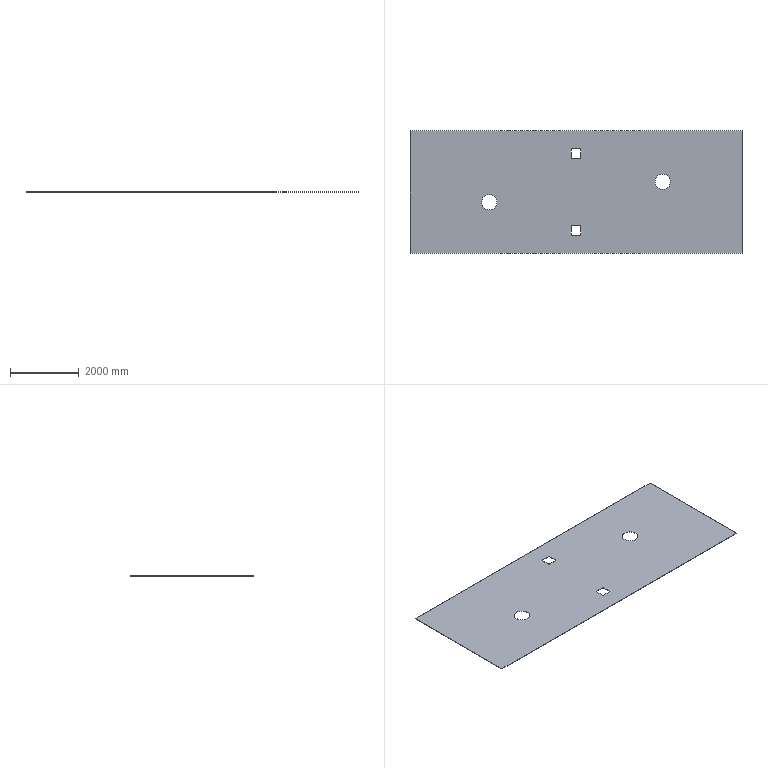Component | SolidWorks | Platform-1 | 1 solid | 26 faces | box 9690 x 3580 x 10 mm | volume 342054589 mm3 | plane 14 | cylinder 12 | commonest cylinder face diameters 60 x8 450 x4 | material Plain Carbon Steel
STEP:
#1=COLOUR_RGB('',0.7922,0.8196,0.9333);
#2=FILL_AREA_STYLE_COLOUR('',#1);
#3=FILL_AREA_STYLE('',(#2));
#4=SURFACE_STYLE_FILL_AREA(#3);
#5=SURFACE_SIDE_STYLE('',(#4));
#6=SURFACE_STYLE_USAGE(.BOTH.,#5);
#7=PRESENTATION_STYLE_ASSIGNMENT((#6));
#8=CARTESIAN_POINT('',(157.197,66.784,219.527));
#9=VERTEX_POINT('',#8);
#10=CARTESIAN_POINT('',(157.197,49.068,219.527));
#11=VERTEX_POINT('',#10);
#12=CARTESIAN_POINT('',(157.197,57.926,219.527));
#13=DIRECTION('',(0.,-0.,1.));
#14=DIRECTION('',(0.,-1.,-0.));
#15=AXIS2_PLACEMENT_3D('',#12,#13,#14);
#16=CIRCLE('',#15,8.858);
#17=EDGE_CURVE('',#9,#11,#16,.T.);
#18=ORIENTED_EDGE('',*,*,#17,.F.);
#19=CARTESIAN_POINT('',(157.197,66.784,219.92));
#20=VERTEX_POINT('',#19);
#21=CARTESIAN_POINT('',(157.197,66.784,219.527));
#22=DIRECTION('',(0.,-0.,1.));
#23=VECTOR('',#22,39.37);
#24=LINE('',#21,#23);
#25=EDGE_CURVE('',#9,#20,#24,.T.);
#26=ORIENTED_EDGE('',*,*,#25,.T.);
#27=CARTESIAN_POINT('',(157.197,49.068,219.92));
#28=VERTEX_POINT('',#27);
#29=CARTESIAN_POINT('',(157.197,57.926,219.92));
#30=DIRECTION('',(0.,-0.,1.));
#31=DIRECTION('',(0.,-1.,-0.));
#32=AXIS2_PLACEMENT_3D('',#29,#30,#31);
#33=CIRCLE('',#32,8.858);
#34=EDGE_CURVE('',#20,#28,#33,.T.);
#35=ORIENTED_EDGE('',*,*,#34,.T.);
#36=CARTESIAN_POINT('',(157.197,49.068,219.527));
#37=DIRECTION('',(0.,-0.,1.));
#38=VECTOR('',#37,39.37);
#39=LINE('',#36,#38);
#40=EDGE_CURVE('',#11,#28,#39,.T.);
#41=ORIENTED_EDGE('',*,*,#40,.F.);
#42=EDGE_LOOP('',(#18,#26,#35,#41));
#43=FACE_OUTER_BOUND('',#42,.T.);
#44=CARTESIAN_POINT('',(157.197,57.926,219.527));
#45=DIRECTION('',(0.,-0.,1.));
#46=DIRECTION('',(0.,-1.,-0.));
#47=AXIS2_PLACEMENT_3D('',#44,#45,#46);
#48=CYLINDRICAL_SURFACE('',#47,8.858);
#49=ADVANCED_FACE('',(#43),#48,.F.);
#50=CARTESIAN_POINT('',(-42.016,43.162,219.527));
#51=VERTEX_POINT('',#50);
#52=CARTESIAN_POINT('',(-42.016,25.446,219.527));
#53=VERTEX_POINT('',#52);
#54=CARTESIAN_POINT('',(-42.016,34.304,219.527));
#55=DIRECTION('',(0.,-0.,1.));
#56=DIRECTION('',(0.,-1.,-0.));
#57=AXIS2_PLACEMENT_3D('',#54,#55,#56);
#58=CIRCLE('',#57,8.858);
#59=EDGE_CURVE('',#51,#53,#58,.T.);
#60=ORIENTED_EDGE('',*,*,#59,.F.);
#61=CARTESIAN_POINT('',(-42.016,43.162,219.92));
#62=VERTEX_POINT('',#61);
#63=CARTESIAN_POINT('',(-42.016,43.162,219.527));
#64=DIRECTION('',(0.,-0.,1.));
#65=VECTOR('',#64,39.37);
#66=LINE('',#63,#65);
#67=EDGE_CURVE('',#51,#62,#66,.T.);
#68=ORIENTED_EDGE('',*,*,#67,.T.);
#69=CARTESIAN_POINT('',(-42.016,25.446,219.92));
#70=VERTEX_POINT('',#69);
#71=CARTESIAN_POINT('',(-42.016,34.304,219.92));
#72=DIRECTION('',(0.,-0.,1.));
#73=DIRECTION('',(0.,-1.,-0.));
#74=AXIS2_PLACEMENT_3D('',#71,#72,#73);
#75=CIRCLE('',#74,8.858);
#76=EDGE_CURVE('',#62,#70,#75,.T.);
#77=ORIENTED_EDGE('',*,*,#76,.T.);
#78=CARTESIAN_POINT('',(-42.016,25.446,219.527));
#79=DIRECTION('',(0.,-0.,1.));
#80=VECTOR('',#79,39.37);
#81=LINE('',#78,#80);
#82=EDGE_CURVE('',#53,#70,#81,.T.);
#83=ORIENTED_EDGE('',*,*,#82,.F.);
#84=EDGE_LOOP('',(#60,#68,#77,#83));
#85=FACE_OUTER_BOUND('',#84,.T.);
#86=CARTESIAN_POINT('',(-42.016,34.304,219.527));
#87=DIRECTION('',(0.,-0.,1.));
#88=DIRECTION('',(0.,-1.,-0.));
#89=AXIS2_PLACEMENT_3D('',#86,#87,#88);
#90=CYLINDRICAL_SURFACE('',#89,8.858);
#91=ADVANCED_FACE('',(#85),#90,.F.);
#92=CARTESIAN_POINT('',(248.339,-24.357,219.92));
#93=VERTEX_POINT('',#92);
#94=CARTESIAN_POINT('',(248.339,116.588,219.92));
#95=VERTEX_POINT('',#94);
#96=CARTESIAN_POINT('',(248.339,116.588,219.92));
#97=DIRECTION('',(0.,1.,0.));
#98=VECTOR('',#97,39.37);
#99=LINE('',#96,#98);
#100=EDGE_CURVE('',#93,#95,#99,.T.);
#101=ORIENTED_EDGE('',*,*,#100,.F.);
#102=CARTESIAN_POINT('',(248.339,-24.357,219.527));
#103=VERTEX_POINT('',#102);
#104=CARTESIAN_POINT('',(248.339,-24.357,219.527));
#105=DIRECTION('',(0.,-0.,1.));
#106=VECTOR('',#105,39.37);
#107=LINE('',#104,#106);
#108=EDGE_CURVE('',#103,#93,#107,.T.);
#109=ORIENTED_EDGE('',*,*,#108,.F.);
#110=CARTESIAN_POINT('',(248.339,116.588,219.527));
#111=VERTEX_POINT('',#110);
#112=CARTESIAN_POINT('',(248.339,116.588,219.527));
#113=DIRECTION('',(0.,1.,0.));
#114=VECTOR('',#113,39.37);
#115=LINE('',#112,#114);
#116=EDGE_CURVE('',#103,#111,#115,.T.);
#117=ORIENTED_EDGE('',*,*,#116,.T.);
#118=CARTESIAN_POINT('',(248.339,116.588,219.527));
#119=DIRECTION('',(0.,-0.,1.));
#120=VECTOR('',#119,39.37);
#121=LINE('',#118,#120);
#122=EDGE_CURVE('',#111,#95,#121,.T.);
#123=ORIENTED_EDGE('',*,*,#122,.T.);
#124=EDGE_LOOP('',(#101,#109,#117,#123));
#125=FACE_OUTER_BOUND('',#124,.T.);
#126=CARTESIAN_POINT('',(248.339,116.588,219.527));
#127=DIRECTION('',(1.,0.,0.));
#128=DIRECTION('',(0.,1.,0.));
#129=AXIS2_PLACEMENT_3D('',#126,#127,#128);
#130=PLANE('',#129);
#131=ADVANCED_FACE('',(#125),#130,.T.);
#132=CARTESIAN_POINT('',(-133.157,-24.357,219.92));
#133=VERTEX_POINT('',#132);
#134=CARTESIAN_POINT('',(-133.157,-24.357,219.92));
#135=DIRECTION('',(1.,0.,0.));
#136=VECTOR('',#135,39.37);
#137=LINE('',#134,#136);
#138=EDGE_CURVE('',#133,#93,#137,.T.);
#139=ORIENTED_EDGE('',*,*,#138,.F.);
#140=CARTESIAN_POINT('',(-133.157,-24.357,219.527));
#141=VERTEX_POINT('',#140);
#142=CARTESIAN_POINT('',(-133.157,-24.357,219.527));
#143=DIRECTION('',(0.,-0.,1.));
#144=VECTOR('',#143,39.37);
#145=LINE('',#142,#144);
#146=EDGE_CURVE('',#141,#133,#145,.T.);
#147=ORIENTED_EDGE('',*,*,#146,.F.);
#148=CARTESIAN_POINT('',(-133.157,-24.357,219.527));
#149=DIRECTION('',(1.,0.,0.));
#150=VECTOR('',#149,39.37);
#151=LINE('',#148,#150);
#152=EDGE_CURVE('',#141,#103,#151,.T.);
#153=ORIENTED_EDGE('',*,*,#152,.T.);
#154=ORIENTED_EDGE('',*,*,#108,.T.);
#155=EDGE_LOOP('',(#139,#147,#153,#154));
#156=FACE_OUTER_BOUND('',#155,.T.);
#157=CARTESIAN_POINT('',(-133.157,-24.357,219.527));
#158=DIRECTION('',(0.,-1.,-0.));
#159=DIRECTION('',(1.,0.,0.));
#160=AXIS2_PLACEMENT_3D('',#157,#158,#159);
#161=PLANE('',#160);
#162=ADVANCED_FACE('',(#156),#161,.T.);
#163=CARTESIAN_POINT('',(-133.157,116.588,219.92));
#164=VERTEX_POINT('',#163);
#165=CARTESIAN_POINT('',(-133.157,116.588,219.92));
#166=DIRECTION('',(0.,-1.,-0.));
#167=VECTOR('',#166,39.37);
#168=LINE('',#165,#167);
#169=EDGE_CURVE('',#164,#133,#168,.T.);
#170=ORIENTED_EDGE('',*,*,#169,.F.);
#171=CARTESIAN_POINT('',(-133.157,116.588,219.527));
#172=VERTEX_POINT('',#171);
#173=CARTESIAN_POINT('',(-133.157,116.588,219.527));
#174=DIRECTION('',(0.,-0.,1.));
#175=VECTOR('',#174,39.37);
#176=LINE('',#173,#175);
#177=EDGE_CURVE('',#172,#164,#176,.T.);
#178=ORIENTED_EDGE('',*,*,#177,.F.);
#179=CARTESIAN_POINT('',(-133.157,116.588,219.527));
#180=DIRECTION('',(0.,-1.,-0.));
#181=VECTOR('',#180,39.37);
#182=LINE('',#179,#181);
#183=EDGE_CURVE('',#172,#141,#182,.T.);
#184=ORIENTED_EDGE('',*,*,#183,.T.);
#185=ORIENTED_EDGE('',*,*,#146,.T.);
#186=EDGE_LOOP('',(#170,#178,#184,#185));
#187=FACE_OUTER_BOUND('',#186,.T.);
#188=CARTESIAN_POINT('',(-133.157,116.588,219.527));
#189=DIRECTION('',(-1.,0.,0.));
#190=DIRECTION('',(0.,-1.,-0.));
#191=AXIS2_PLACEMENT_3D('',#188,#189,#190);
#192=PLANE('',#191);
#193=ADVANCED_FACE('',(#187),#192,.T.);
#194=CARTESIAN_POINT('',(-133.157,116.588,219.92));
#195=DIRECTION('',(-1.,0.,0.));
#196=VECTOR('',#195,39.37);
#197=LINE('',#194,#196);
#198=EDGE_CURVE('',#95,#164,#197,.T.);
#199=ORIENTED_EDGE('',*,*,#198,.F.);
#200=ORIENTED_EDGE('',*,*,#122,.F.);
#201=CARTESIAN_POINT('',(-133.157,116.588,219.527));
#202=DIRECTION('',(-1.,0.,0.));
#203=VECTOR('',#202,39.37);
#204=LINE('',#201,#203);
#205=EDGE_CURVE('',#111,#172,#204,.T.);
#206=ORIENTED_EDGE('',*,*,#205,.T.);
#207=ORIENTED_EDGE('',*,*,#177,.T.);
#208=EDGE_LOOP('',(#199,#200,#206,#207));
#209=FACE_OUTER_BOUND('',#208,.T.);
#210=CARTESIAN_POINT('',(-133.157,116.588,219.527));
#211=DIRECTION('',(0.,1.,0.));
#212=DIRECTION('',(-1.,0.,0.));
#213=AXIS2_PLACEMENT_3D('',#210,#211,#212);
#214=PLANE('',#213);
#215=ADVANCED_FACE('',(#209),#214,.T.);
#216=CARTESIAN_POINT('',(62.118,7.926,219.527));
#217=VERTEX_POINT('',#216);
#218=CARTESIAN_POINT('',(53.063,7.926,219.527));
#219=VERTEX_POINT('',#218);
#220=CARTESIAN_POINT('',(53.063,7.926,219.527));
#221=DIRECTION('',(-1.,0.,0.));
#222=VECTOR('',#221,39.37);
#223=LINE('',#220,#222);
#224=EDGE_CURVE('',#217,#219,#223,.T.);
#225=ORIENTED_EDGE('',*,*,#224,.T.);
#226=CARTESIAN_POINT('',(51.882,6.745,219.527));
#227=VERTEX_POINT('',#226);
#228=CARTESIAN_POINT('',(53.063,6.745,219.527));
#229=DIRECTION('',(0.,-0.,1.));
#230=DIRECTION('',(0.,1.,0.));
#231=AXIS2_PLACEMENT_3D('',#228,#229,#230);
#232=CIRCLE('',#231,1.181);
#233=EDGE_CURVE('',#219,#227,#232,.T.);
#234=ORIENTED_EDGE('',*,*,#233,.T.);
#235=CARTESIAN_POINT('',(51.882,-2.31,219.527));
#236=VERTEX_POINT('',#235);
#237=CARTESIAN_POINT('',(51.882,-2.31,219.527));
#238=DIRECTION('',(-0.,-1.,-0.));
#239=VECTOR('',#238,39.37);
#240=LINE('',#237,#239);
#241=EDGE_CURVE('',#227,#236,#240,.T.);
#242=ORIENTED_EDGE('',*,*,#241,.T.);
#243=CARTESIAN_POINT('',(53.063,-3.491,219.527));
#244=VERTEX_POINT('',#243);
#245=CARTESIAN_POINT('',(53.063,-2.31,219.527));
#246=DIRECTION('',(0.,-0.,1.));
#247=DIRECTION('',(0.,1.,0.));
#248=AXIS2_PLACEMENT_3D('',#245,#246,#247);
#249=CIRCLE('',#248,1.181);
#250=EDGE_CURVE('',#236,#244,#249,.T.);
#251=ORIENTED_EDGE('',*,*,#250,.T.);
#252=CARTESIAN_POINT('',(62.118,-3.491,219.527));
#253=VERTEX_POINT('',#252);
#254=CARTESIAN_POINT('',(53.063,-3.491,219.527));
#255=DIRECTION('',(1.,0.,0.));
#256=VECTOR('',#255,39.37);
#257=LINE('',#254,#256);
#258=EDGE_CURVE('',#244,#253,#257,.T.);
#259=ORIENTED_EDGE('',*,*,#258,.T.);
#260=CARTESIAN_POINT('',(63.299,-2.31,219.527));
#261=VERTEX_POINT('',#260);
#262=CARTESIAN_POINT('',(62.118,-2.31,219.527));
#263=DIRECTION('',(0.,-0.,1.));
#264=DIRECTION('',(0.,-1.,0.));
#265=AXIS2_PLACEMENT_3D('',#262,#263,#264);
#266=CIRCLE('',#265,1.181);
#267=EDGE_CURVE('',#253,#261,#266,.T.);
#268=ORIENTED_EDGE('',*,*,#267,.T.);
#269=CARTESIAN_POINT('',(63.299,6.745,219.527));
#270=VERTEX_POINT('',#269);
#271=CARTESIAN_POINT('',(63.299,-2.31,219.527));
#272=DIRECTION('',(0.,1.,0.));
#273=VECTOR('',#272,39.37);
#274=LINE('',#271,#273);
#275=EDGE_CURVE('',#261,#270,#274,.T.);
#276=ORIENTED_EDGE('',*,*,#275,.T.);
#277=CARTESIAN_POINT('',(62.118,6.745,219.527));
#278=DIRECTION('',(0.,-0.,1.));
#279=DIRECTION('',(0.,1.,0.));
#280=AXIS2_PLACEMENT_3D('',#277,#278,#279);
#281=CIRCLE('',#280,1.181);
#282=EDGE_CURVE('',#270,#217,#281,.T.);
#283=ORIENTED_EDGE('',*,*,#282,.T.);
#284=EDGE_LOOP('',(#225,#234,#242,#251,#259,#268,#276,#283));
#285=FACE_BOUND('',#284,.T.);
#286=CARTESIAN_POINT('',(51.882,94.54,219.527));
#287=VERTEX_POINT('',#286);
#288=CARTESIAN_POINT('',(51.882,85.485,219.527));
#289=VERTEX_POINT('',#288);
#290=CARTESIAN_POINT('',(51.882,94.54,219.527));
#291=DIRECTION('',(0.,-1.,-0.));
#292=VECTOR('',#291,39.37);
#293=LINE('',#290,#292);
#294=EDGE_CURVE('',#287,#289,#293,.T.);
#295=ORIENTED_EDGE('',*,*,#294,.T.);
#296=CARTESIAN_POINT('',(53.063,84.304,219.527));
#297=VERTEX_POINT('',#296);
#298=CARTESIAN_POINT('',(53.063,85.485,219.527));
#299=DIRECTION('',(0.,-0.,1.));
#300=DIRECTION('',(0.,-1.,0.));
#301=AXIS2_PLACEMENT_3D('',#298,#299,#300);
#302=CIRCLE('',#301,1.181);
#303=EDGE_CURVE('',#289,#297,#302,.T.);
#304=ORIENTED_EDGE('',*,*,#303,.T.);
#305=CARTESIAN_POINT('',(62.118,84.304,219.527));
#306=VERTEX_POINT('',#305);
#307=CARTESIAN_POINT('',(53.063,84.304,219.527));
#308=DIRECTION('',(1.,0.,0.));
#309=VECTOR('',#308,39.37);
#310=LINE('',#307,#309);
#311=EDGE_CURVE('',#297,#306,#310,.T.);
#312=ORIENTED_EDGE('',*,*,#311,.T.);
#313=CARTESIAN_POINT('',(63.299,85.485,219.527));
#314=VERTEX_POINT('',#313);
#315=CARTESIAN_POINT('',(62.118,85.485,219.527));
#316=DIRECTION('',(0.,-0.,1.));
#317=DIRECTION('',(0.,-1.,0.));
#318=AXIS2_PLACEMENT_3D('',#315,#316,#317);
#319=CIRCLE('',#318,1.181);
#320=EDGE_CURVE('',#306,#314,#319,.T.);
#321=ORIENTED_EDGE('',*,*,#320,.T.);
#322=CARTESIAN_POINT('',(63.299,94.54,219.527));
#323=VERTEX_POINT('',#322);
#324=CARTESIAN_POINT('',(63.299,94.54,219.527));
#325=DIRECTION('',(-0.,1.,0.));
#326=VECTOR('',#325,39.37);
#327=LINE('',#324,#326);
#328=EDGE_CURVE('',#314,#323,#327,.T.);
#329=ORIENTED_EDGE('',*,*,#328,.T.);
#330=CARTESIAN_POINT('',(62.118,95.721,219.527));
#331=VERTEX_POINT('',#330);
#332=CARTESIAN_POINT('',(62.118,94.54,219.527));
#333=DIRECTION('',(0.,-0.,1.));
#334=DIRECTION('',(0.,1.,0.));
#335=AXIS2_PLACEMENT_3D('',#332,#333,#334);
#336=CIRCLE('',#335,1.181);
#337=EDGE_CURVE('',#323,#331,#336,.T.);
#338=ORIENTED_EDGE('',*,*,#337,.T.);
#339=CARTESIAN_POINT('',(53.063,95.721,219.527));
#340=VERTEX_POINT('',#339);
#341=CARTESIAN_POINT('',(53.063,95.721,219.527));
#342=DIRECTION('',(-1.,0.,0.));
#343=VECTOR('',#342,39.37);
#344=LINE('',#341,#343);
#345=EDGE_CURVE('',#331,#340,#344,.T.);
#346=ORIENTED_EDGE('',*,*,#345,.T.);
#347=CARTESIAN_POINT('',(53.063,94.54,219.527));
#348=DIRECTION('',(0.,-0.,1.));
#349=DIRECTION('',(0.,-1.,0.));
#350=AXIS2_PLACEMENT_3D('',#347,#348,#349);
#351=CIRCLE('',#350,1.181);
#352=EDGE_CURVE('',#340,#287,#351,.T.);
#353=ORIENTED_EDGE('',*,*,#352,.T.);
#354=EDGE_LOOP('',(#295,#304,#312,#321,#329,#338,#346,#353));
#355=FACE_BOUND('',#354,.T.);
#356=CARTESIAN_POINT('',(157.197,57.926,219.527));
#357=DIRECTION('',(0.,-0.,1.));
#358=DIRECTION('',(0.,-1.,-0.));
#359=AXIS2_PLACEMENT_3D('',#356,#357,#358);
#360=CIRCLE('',#359,8.858);
#361=EDGE_CURVE('',#11,#9,#360,.T.);
#362=ORIENTED_EDGE('',*,*,#361,.T.);
#363=ORIENTED_EDGE('',*,*,#17,.T.);
#364=EDGE_LOOP('',(#362,#363));
#365=FACE_BOUND('',#364,.T.);
#366=CARTESIAN_POINT('',(-42.016,34.304,219.527));
#367=DIRECTION('',(0.,-0.,1.));
#368=DIRECTION('',(0.,-1.,-0.));
#369=AXIS2_PLACEMENT_3D('',#366,#367,#368);
#370=CIRCLE('',#369,8.858);
#371=EDGE_CURVE('',#53,#51,#370,.T.);
#372=ORIENTED_EDGE('',*,*,#371,.T.);
#373=ORIENTED_EDGE('',*,*,#59,.T.);
#374=EDGE_LOOP('',(#372,#373));
#375=FACE_BOUND('',#374,.T.);
#376=ORIENTED_EDGE('',*,*,#116,.F.);
#377=ORIENTED_EDGE('',*,*,#152,.F.);
#378=ORIENTED_EDGE('',*,*,#183,.F.);
#379=ORIENTED_EDGE('',*,*,#205,.F.);
#380=EDGE_LOOP('',(#376,#377,#378,#379));
#381=FACE_OUTER_BOUND('',#380,.T.);
#382=CARTESIAN_POINT('',(57.591,46.115,219.527));
#383=DIRECTION('',(0.,-0.,1.));
#384=DIRECTION('',(0.,-1.,-0.));
#385=AXIS2_PLACEMENT_3D('',#382,#383,#384);
#386=PLANE('',#385);
#387=ADVANCED_FACE('',(#285,#355,#365,#375,#381),#386,.F.);
#388=CARTESIAN_POINT('',(53.063,7.926,219.92));
#389=VERTEX_POINT('',#388);
#390=CARTESIAN_POINT('',(51.882,6.745,219.92));
#391=VERTEX_POINT('',#390);
#392=CARTESIAN_POINT('',(53.063,6.745,219.92));
#393=DIRECTION('',(0.,-0.,1.));
#394=DIRECTION('',(0.,1.,0.));
#395=AXIS2_PLACEMENT_3D('',#392,#393,#394);
#396=CIRCLE('',#395,1.181);
#397=EDGE_CURVE('',#389,#391,#396,.T.);
#398=ORIENTED_EDGE('',*,*,#397,.F.);
#399=CARTESIAN_POINT('',(62.118,7.926,219.92));
#400=VERTEX_POINT('',#399);
#401=CARTESIAN_POINT('',(53.063,7.926,219.92));
#402=DIRECTION('',(-1.,0.,0.));
#403=VECTOR('',#402,39.37);
#404=LINE('',#401,#403);
#405=EDGE_CURVE('',#400,#389,#404,.T.);
#406=ORIENTED_EDGE('',*,*,#405,.F.);
#407=CARTESIAN_POINT('',(63.299,6.745,219.92));
#408=VERTEX_POINT('',#407);
#409=CARTESIAN_POINT('',(62.118,6.745,219.92));
#410=DIRECTION('',(0.,-0.,1.));
#411=DIRECTION('',(0.,1.,0.));
#412=AXIS2_PLACEMENT_3D('',#409,#410,#411);
#413=CIRCLE('',#412,1.181);
#414=EDGE_CURVE('',#408,#400,#413,.T.);
#415=ORIENTED_EDGE('',*,*,#414,.F.);
#416=CARTESIAN_POINT('',(63.299,-2.31,219.92));
#417=VERTEX_POINT('',#416);
#418=CARTESIAN_POINT('',(63.299,-2.31,219.92));
#419=DIRECTION('',(0.,1.,0.));
#420=VECTOR('',#419,39.37);
#421=LINE('',#418,#420);
#422=EDGE_CURVE('',#417,#408,#421,.T.);
#423=ORIENTED_EDGE('',*,*,#422,.F.);
#424=CARTESIAN_POINT('',(62.118,-3.491,219.92));
#425=VERTEX_POINT('',#424);
#426=CARTESIAN_POINT('',(62.118,-2.31,219.92));
#427=DIRECTION('',(0.,-0.,1.));
#428=DIRECTION('',(0.,-1.,0.));
#429=AXIS2_PLACEMENT_3D('',#426,#427,#428);
#430=CIRCLE('',#429,1.181);
#431=EDGE_CURVE('',#425,#417,#430,.T.);
#432=ORIENTED_EDGE('',*,*,#431,.F.);
#433=CARTESIAN_POINT('',(53.063,-3.491,219.92));
#434=VERTEX_POINT('',#433);
#435=CARTESIAN_POINT('',(53.063,-3.491,219.92));
#436=DIRECTION('',(1.,0.,0.));
#437=VECTOR('',#436,39.37);
#438=LINE('',#435,#437);
#439=EDGE_CURVE('',#434,#425,#438,.T.);
#440=ORIENTED_EDGE('',*,*,#439,.F.);
#441=CARTESIAN_POINT('',(51.882,-2.31,219.92));
#442=VERTEX_POINT('',#441);
#443=CARTESIAN_POINT('',(53.063,-2.31,219.92));
#444=DIRECTION('',(0.,-0.,1.));
#445=DIRECTION('',(0.,1.,0.));
#446=AXIS2_PLACEMENT_3D('',#443,#444,#445);
#447=CIRCLE('',#446,1.181);
#448=EDGE_CURVE('',#442,#434,#447,.T.);
#449=ORIENTED_EDGE('',*,*,#448,.F.);
#450=CARTESIAN_POINT('',(51.882,-2.31,219.92));
#451=DIRECTION('',(-0.,-1.,-0.));
#452=VECTOR('',#451,39.37);
#453=LINE('',#450,#452);
#454=EDGE_CURVE('',#391,#442,#453,.T.);
#455=ORIENTED_EDGE('',*,*,#454,.F.);
#456=EDGE_LOOP('',(#398,#406,#415,#423,#432,#440,#449,#455));
#457=FACE_BOUND('',#456,.T.);
#458=CARTESIAN_POINT('',(51.882,85.485,219.92));
#459=VERTEX_POINT('',#458);
#460=CARTESIAN_POINT('',(53.063,84.304,219.92));
#461=VERTEX_POINT('',#460);
#462=CARTESIAN_POINT('',(53.063,85.485,219.92));
#463=DIRECTION('',(0.,-0.,1.));
#464=DIRECTION('',(0.,-1.,0.));
#465=AXIS2_PLACEMENT_3D('',#462,#463,#464);
#466=CIRCLE('',#465,1.181);
#467=EDGE_CURVE('',#459,#461,#466,.T.);
#468=ORIENTED_EDGE('',*,*,#467,.F.);
#469=CARTESIAN_POINT('',(51.882,94.54,219.92));
#470=VERTEX_POINT('',#469);
#471=CARTESIAN_POINT('',(51.882,94.54,219.92));
#472=DIRECTION('',(0.,-1.,-0.));
#473=VECTOR('',#472,39.37);
#474=LINE('',#471,#473);
#475=EDGE_CURVE('',#470,#459,#474,.T.);
#476=ORIENTED_EDGE('',*,*,#475,.F.);
#477=CARTESIAN_POINT('',(53.063,95.721,219.92));
#478=VERTEX_POINT('',#477);
#479=CARTESIAN_POINT('',(53.063,94.54,219.92));
#480=DIRECTION('',(0.,-0.,1.));
#481=DIRECTION('',(0.,-1.,0.));
#482=AXIS2_PLACEMENT_3D('',#479,#480,#481);
#483=CIRCLE('',#482,1.181);
#484=EDGE_CURVE('',#478,#470,#483,.T.);
#485=ORIENTED_EDGE('',*,*,#484,.F.);
#486=CARTESIAN_POINT('',(62.118,95.721,219.92));
#487=VERTEX_POINT('',#486);
#488=CARTESIAN_POINT('',(53.063,95.721,219.92));
#489=DIRECTION('',(-1.,0.,0.));
#490=VECTOR('',#489,39.37);
#491=LINE('',#488,#490);
#492=EDGE_CURVE('',#487,#478,#491,.T.);
#493=ORIENTED_EDGE('',*,*,#492,.F.);
#494=CARTESIAN_POINT('',(63.299,94.54,219.92));
#495=VERTEX_POINT('',#494);
#496=CARTESIAN_POINT('',(62.118,94.54,219.92));
#497=DIRECTION('',(0.,-0.,1.));
#498=DIRECTION('',(0.,1.,0.));
#499=AXIS2_PLACEMENT_3D('',#496,#497,#498);
#500=CIRCLE('',#499,1.181);
#501=EDGE_CURVE('',#495,#487,#500,.T.);
#502=ORIENTED_EDGE('',*,*,#501,.F.);
#503=CARTESIAN_POINT('',(63.299,85.485,219.92));
#504=VERTEX_POINT('',#503);
#505=CARTESIAN_POINT('',(63.299,94.54,219.92));
#506=DIRECTION('',(-0.,1.,0.));
#507=VECTOR('',#506,39.37);
#508=LINE('',#505,#507);
#509=EDGE_CURVE('',#504,#495,#508,.T.);
#510=ORIENTED_EDGE('',*,*,#509,.F.);
#511=CARTESIAN_POINT('',(62.118,84.304,219.92));
#512=VERTEX_POINT('',#511);
#513=CARTESIAN_POINT('',(62.118,85.485,219.92));
#514=DIRECTION('',(0.,-0.,1.));
#515=DIRECTION('',(0.,-1.,0.));
#516=AXIS2_PLACEMENT_3D('',#513,#514,#515);
#517=CIRCLE('',#516,1.181);
#518=EDGE_CURVE('',#512,#504,#517,.T.);
#519=ORIENTED_EDGE('',*,*,#518,.F.);
#520=CARTESIAN_POINT('',(53.063,84.304,219.92));
#521=DIRECTION('',(1.,0.,0.));
#522=VECTOR('',#521,39.37);
#523=LINE('',#520,#522);
#524=EDGE_CURVE('',#461,#512,#523,.T.);
#525=ORIENTED_EDGE('',*,*,#524,.F.);
#526=EDGE_LOOP('',(#468,#476,#485,#493,#502,#510,#519,#525));
#527=FACE_BOUND('',#526,.T.);
#528=CARTESIAN_POINT('',(157.197,57.926,219.92));
#529=DIRECTION('',(0.,-0.,1.));
#530=DIRECTION('',(0.,-1.,-0.));
#531=AXIS2_PLACEMENT_3D('',#528,#529,#530);
#532=CIRCLE('',#531,8.858);
#533=EDGE_CURVE('',#28,#20,#532,.T.);
#534=ORIENTED_EDGE('',*,*,#533,.F.);
#535=ORIENTED_EDGE('',*,*,#34,.F.);
#536=EDGE_LOOP('',(#534,#535));
#537=FACE_BOUND('',#536,.T.);
#538=CARTESIAN_POINT('',(-42.016,34.304,219.92));
#539=DIRECTION('',(0.,-0.,1.));
#540=DIRECTION('',(0.,-1.,-0.));
#541=AXIS2_PLACEMENT_3D('',#538,#539,#540);
#542=CIRCLE('',#541,8.858);
#543=EDGE_CURVE('',#70,#62,#542,.T.);
#544=ORIENTED_EDGE('',*,*,#543,.F.);
#545=ORIENTED_EDGE('',*,*,#76,.F.);
#546=EDGE_LOOP('',(#544,#545));
#547=FACE_BOUND('',#546,.T.);
#548=ORIENTED_EDGE('',*,*,#100,.T.);
#549=ORIENTED_EDGE('',*,*,#198,.T.);
#550=ORIENTED_EDGE('',*,*,#169,.T.);
#551=ORIENTED_EDGE('',*,*,#138,.T.);
#552=EDGE_LOOP('',(#548,#549,#550,#551));
#553=FACE_OUTER_BOUND('',#552,.T.);
#554=CARTESIAN_POINT('',(57.591,46.115,219.92));
#555=DIRECTION('',(0.,-0.,1.));
#556=DIRECTION('',(0.,-1.,-0.));
#557=AXIS2_PLACEMENT_3D('',#554,#555,#556);
#558=PLANE('',#557);
#559=ADVANCED_FACE('',(#457,#527,#537,#547,#553),#558,.T.);
#560=ORIENTED_EDGE('',*,*,#67,.F.);
#561=ORIENTED_EDGE('',*,*,#371,.F.);
#562=ORIENTED_EDGE('',*,*,#82,.T.);
#563=ORIENTED_EDGE('',*,*,#543,.T.);
#564=EDGE_LOOP('',(#560,#561,#562,#563));
#565=FACE_OUTER_BOUND('',#564,.T.);
#566=CARTESIAN_POINT('',(-42.016,34.304,219.527));
#567=DIRECTION('',(0.,-0.,1.));
#568=DIRECTION('',(0.,-1.,-0.));
#569=AXIS2_PLACEMENT_3D('',#566,#567,#568);
#570=CYLINDRICAL_SURFACE('',#569,8.858);
#571=ADVANCED_FACE('',(#565),#570,.F.);
#572=ORIENTED_EDGE('',*,*,#25,.F.);
#573=ORIENTED_EDGE('',*,*,#361,.F.);
#574=ORIENTED_EDGE('',*,*,#40,.T.);
#575=ORIENTED_EDGE('',*,*,#533,.T.);
#576=EDGE_LOOP('',(#572,#573,#574,#575));
#577=FACE_OUTER_BOUND('',#576,.T.);
#578=CARTESIAN_POINT('',(157.197,57.926,219.527));
#579=DIRECTION('',(0.,-0.,1.));
#580=DIRECTION('',(0.,-1.,-0.));
#581=AXIS2_PLACEMENT_3D('',#578,#579,#580);
#582=CYLINDRICAL_SURFACE('',#581,8.858);
#583=ADVANCED_FACE('',(#577),#582,.F.);
#584=ORIENTED_EDGE('',*,*,#467,.T.);
#585=CARTESIAN_POINT('',(53.063,84.304,219.527));
#586=DIRECTION('',(0.,-0.,1.));
#587=VECTOR('',#586,39.37);
#588=LINE('',#585,#587);
#589=EDGE_CURVE('',#297,#461,#588,.T.);
#590=ORIENTED_EDGE('',*,*,#589,.F.);
#591=ORIENTED_EDGE('',*,*,#303,.F.);
#592=CARTESIAN_POINT('',(51.882,85.485,219.527));
#593=DIRECTION('',(0.,-0.,1.));
#594=VECTOR('',#593,39.37);
#595=LINE('',#592,#594);
#596=EDGE_CURVE('',#289,#459,#595,.T.);
#597=ORIENTED_EDGE('',*,*,#596,.T.);
#598=EDGE_LOOP('',(#584,#590,#591,#597));
#599=FACE_OUTER_BOUND('',#598,.T.);
#600=CARTESIAN_POINT('',(53.063,85.485,219.527));
#601=DIRECTION('',(0.,-0.,1.));
#602=DIRECTION('',(0.,-1.,0.));
#603=AXIS2_PLACEMENT_3D('',#600,#601,#602);
#604=CYLINDRICAL_SURFACE('',#603,1.181);
#605=ADVANCED_FACE('',(#599),#604,.F.);
#606=ORIENTED_EDGE('',*,*,#475,.T.);
#607=ORIENTED_EDGE('',*,*,#596,.F.);
#608=ORIENTED_EDGE('',*,*,#294,.F.);
#609=CARTESIAN_POINT('',(51.882,94.54,219.527));
#610=DIRECTION('',(0.,-0.,1.));
#611=VECTOR('',#610,39.37);
#612=LINE('',#609,#611);
#613=EDGE_CURVE('',#287,#470,#612,.T.);
#614=ORIENTED_EDGE('',*,*,#613,.T.);
#615=EDGE_LOOP('',(#606,#607,#608,#614));
#616=FACE_OUTER_BOUND('',#615,.T.);
#617=CARTESIAN_POINT('',(51.882,94.54,219.527));
#618=DIRECTION('',(-1.,-0.,-0.));
#619=DIRECTION('',(0.,-1.,-0.));
#620=AXIS2_PLACEMENT_3D('',#617,#618,#619);
#621=PLANE('',#620);
#622=ADVANCED_FACE('',(#616),#621,.F.);
#623=ORIENTED_EDGE('',*,*,#484,.T.);
#624=ORIENTED_EDGE('',*,*,#613,.F.);
#625=ORIENTED_EDGE('',*,*,#352,.F.);
#626=CARTESIAN_POINT('',(53.063,95.721,219.527));
#627=DIRECTION('',(0.,-0.,1.));
#628=VECTOR('',#627,39.37);
#629=LINE('',#626,#628);
#630=EDGE_CURVE('',#340,#478,#629,.T.);
#631=ORIENTED_EDGE('',*,*,#630,.T.);
#632=EDGE_LOOP('',(#623,#624,#625,#631));
#633=FACE_OUTER_BOUND('',#632,.T.);
#634=CARTESIAN_POINT('',(53.063,94.54,219.527));
#635=DIRECTION('',(0.,-0.,1.));
#636=DIRECTION('',(0.,-1.,0.));
#637=AXIS2_PLACEMENT_3D('',#634,#635,#636);
#638=CYLINDRICAL_SURFACE('',#637,1.181);
#639=ADVANCED_FACE('',(#633),#638,.F.);
#640=ORIENTED_EDGE('',*,*,#492,.T.);
#641=ORIENTED_EDGE('',*,*,#630,.F.);
#642=ORIENTED_EDGE('',*,*,#345,.F.);
#643=CARTESIAN_POINT('',(62.118,95.721,219.527));
#644=DIRECTION('',(0.,-0.,1.));
#645=VECTOR('',#644,39.37);
#646=LINE('',#643,#645);
#647=EDGE_CURVE('',#331,#487,#646,.T.);
#648=ORIENTED_EDGE('',*,*,#647,.T.);
#649=EDGE_LOOP('',(#640,#641,#642,#648));
#650=FACE_OUTER_BOUND('',#649,.T.);
#651=CARTESIAN_POINT('',(53.063,95.721,219.527));
#652=DIRECTION('',(0.,1.,0.));
#653=DIRECTION('',(-1.,0.,0.));
#654=AXIS2_PLACEMENT_3D('',#651,#652,#653);
#655=PLANE('',#654);
#656=ADVANCED_FACE('',(#650),#655,.F.);
#657=ORIENTED_EDGE('',*,*,#501,.T.);
#658=ORIENTED_EDGE('',*,*,#647,.F.);
#659=ORIENTED_EDGE('',*,*,#337,.F.);
#660=CARTESIAN_POINT('',(63.299,94.54,219.527));
#661=DIRECTION('',(0.,-0.,1.));
#662=VECTOR('',#661,39.37);
#663=LINE('',#660,#662);
#664=EDGE_CURVE('',#323,#495,#663,.T.);
#665=ORIENTED_EDGE('',*,*,#664,.T.);
#666=EDGE_LOOP('',(#657,#658,#659,#665));
#667=FACE_OUTER_BOUND('',#666,.T.);
#668=CARTESIAN_POINT('',(62.118,94.54,219.527));
#669=DIRECTION('',(0.,-0.,1.));
#670=DIRECTION('',(0.,-1.,0.));
#671=AXIS2_PLACEMENT_3D('',#668,#669,#670);
#672=CYLINDRICAL_SURFACE('',#671,1.181);
#673=ADVANCED_FACE('',(#667),#672,.F.);
#674=ORIENTED_EDGE('',*,*,#509,.T.);
#675=ORIENTED_EDGE('',*,*,#664,.F.);
#676=ORIENTED_EDGE('',*,*,#328,.F.);
#677=CARTESIAN_POINT('',(63.299,85.485,219.527));
#678=DIRECTION('',(0.,-0.,1.));
#679=VECTOR('',#678,39.37);
#680=LINE('',#677,#679);
#681=EDGE_CURVE('',#314,#504,#680,.T.);
#682=ORIENTED_EDGE('',*,*,#681,.T.);
#683=EDGE_LOOP('',(#674,#675,#676,#682));
#684=FACE_OUTER_BOUND('',#683,.T.);
#685=CARTESIAN_POINT('',(63.299,94.54,219.527));
#686=DIRECTION('',(1.,0.,0.));
#687=DIRECTION('',(-0.,1.,0.));
#688=AXIS2_PLACEMENT_3D('',#685,#686,#687);
#689=PLANE('',#688);
#690=ADVANCED_FACE('',(#684),#689,.F.);
#691=ORIENTED_EDGE('',*,*,#518,.T.);
#692=ORIENTED_EDGE('',*,*,#681,.F.);
#693=ORIENTED_EDGE('',*,*,#320,.F.);
#694=CARTESIAN_POINT('',(62.118,84.304,219.527));
#695=DIRECTION('',(0.,-0.,1.));
#696=VECTOR('',#695,39.37);
#697=LINE('',#694,#696);
#698=EDGE_CURVE('',#306,#512,#697,.T.);
#699=ORIENTED_EDGE('',*,*,#698,.T.);
#700=EDGE_LOOP('',(#691,#692,#693,#699));
#701=FACE_OUTER_BOUND('',#700,.T.);
#702=CARTESIAN_POINT('',(62.118,85.485,219.527));
#703=DIRECTION('',(0.,-0.,1.));
#704=DIRECTION('',(0.,-1.,0.));
#705=AXIS2_PLACEMENT_3D('',#702,#703,#704);
#706=CYLINDRICAL_SURFACE('',#705,1.181);
#707=ADVANCED_FACE('',(#701),#706,.F.);
#708=ORIENTED_EDGE('',*,*,#524,.T.);
#709=ORIENTED_EDGE('',*,*,#698,.F.);
#710=ORIENTED_EDGE('',*,*,#311,.F.);
#711=ORIENTED_EDGE('',*,*,#589,.T.);
#712=EDGE_LOOP('',(#708,#709,#710,#711));
#713=FACE_OUTER_BOUND('',#712,.T.);
#714=CARTESIAN_POINT('',(53.063,84.304,219.527));
#715=DIRECTION('',(0.,-1.,-0.));
#716=DIRECTION('',(1.,0.,0.));
#717=AXIS2_PLACEMENT_3D('',#714,#715,#716);
#718=PLANE('',#717);
#719=ADVANCED_FACE('',(#713),#718,.F.);
#720=ORIENTED_EDGE('',*,*,#397,.T.);
#721=CARTESIAN_POINT('',(51.882,6.745,219.527));
#722=DIRECTION('',(0.,-0.,1.));
#723=VECTOR('',#722,39.37);
#724=LINE('',#721,#723);
#725=EDGE_CURVE('',#227,#391,#724,.T.);
#726=ORIENTED_EDGE('',*,*,#725,.F.);
#727=ORIENTED_EDGE('',*,*,#233,.F.);
#728=CARTESIAN_POINT('',(53.063,7.926,219.527));
#729=DIRECTION('',(0.,-0.,1.));
#730=VECTOR('',#729,39.37);
#731=LINE('',#728,#730);
#732=EDGE_CURVE('',#219,#389,#731,.T.);
#733=ORIENTED_EDGE('',*,*,#732,.T.);
#734=EDGE_LOOP('',(#720,#726,#727,#733));
#735=FACE_OUTER_BOUND('',#734,.T.);
#736=CARTESIAN_POINT('',(53.063,6.745,219.527));
#737=DIRECTION('',(0.,-0.,1.));
#738=DIRECTION('',(0.,-1.,0.));
#739=AXIS2_PLACEMENT_3D('',#736,#737,#738);
#740=CYLINDRICAL_SURFACE('',#739,1.181);
#741=ADVANCED_FACE('',(#735),#740,.F.);
#742=ORIENTED_EDGE('',*,*,#405,.T.);
#743=ORIENTED_EDGE('',*,*,#732,.F.);
#744=ORIENTED_EDGE('',*,*,#224,.F.);
#745=CARTESIAN_POINT('',(62.118,7.926,219.527));
#746=DIRECTION('',(0.,-0.,1.));
#747=VECTOR('',#746,39.37);
#748=LINE('',#745,#747);
#749=EDGE_CURVE('',#217,#400,#748,.T.);
#750=ORIENTED_EDGE('',*,*,#749,.T.);
#751=EDGE_LOOP('',(#742,#743,#744,#750));
#752=FACE_OUTER_BOUND('',#751,.T.);
#753=CARTESIAN_POINT('',(53.063,7.926,219.527));
#754=DIRECTION('',(0.,1.,0.));
#755=DIRECTION('',(-1.,0.,0.));
#756=AXIS2_PLACEMENT_3D('',#753,#754,#755);
#757=PLANE('',#756);
#758=ADVANCED_FACE('',(#752),#757,.F.);
#759=ORIENTED_EDGE('',*,*,#414,.T.);
#760=ORIENTED_EDGE('',*,*,#749,.F.);
#761=ORIENTED_EDGE('',*,*,#282,.F.);
#762=CARTESIAN_POINT('',(63.299,6.745,219.527));
#763=DIRECTION('',(0.,-0.,1.));
#764=VECTOR('',#763,39.37);
#765=LINE('',#762,#764);
#766=EDGE_CURVE('',#270,#408,#765,.T.);
#767=ORIENTED_EDGE('',*,*,#766,.T.);
#768=EDGE_LOOP('',(#759,#760,#761,#767));
#769=FACE_OUTER_BOUND('',#768,.T.);
#770=CARTESIAN_POINT('',(62.118,6.745,219.527));
#771=DIRECTION('',(0.,-0.,1.));
#772=DIRECTION('',(0.,-1.,0.));
#773=AXIS2_PLACEMENT_3D('',#770,#771,#772);
#774=CYLINDRICAL_SURFACE('',#773,1.181);
#775=ADVANCED_FACE('',(#769),#774,.F.);
#776=ORIENTED_EDGE('',*,*,#422,.T.);
#777=ORIENTED_EDGE('',*,*,#766,.F.);
#778=ORIENTED_EDGE('',*,*,#275,.F.);
#779=CARTESIAN_POINT('',(63.299,-2.31,219.527));
#780=DIRECTION('',(0.,-0.,1.));
#781=VECTOR('',#780,39.37);
#782=LINE('',#779,#781);
#783=EDGE_CURVE('',#261,#417,#782,.T.);
#784=ORIENTED_EDGE('',*,*,#783,.T.);
#785=EDGE_LOOP('',(#776,#777,#778,#784));
#786=FACE_OUTER_BOUND('',#785,.T.);
#787=CARTESIAN_POINT('',(63.299,-2.31,219.527));
#788=DIRECTION('',(1.,-0.,-0.));
#789=DIRECTION('',(0.,1.,0.));
#790=AXIS2_PLACEMENT_3D('',#787,#788,#789);
#791=PLANE('',#790);
#792=ADVANCED_FACE('',(#786),#791,.F.);
#793=ORIENTED_EDGE('',*,*,#431,.T.);
#794=ORIENTED_EDGE('',*,*,#783,.F.);
#795=ORIENTED_EDGE('',*,*,#267,.F.);
#796=CARTESIAN_POINT('',(62.118,-3.491,219.527));
#797=DIRECTION('',(0.,-0.,1.));
#798=VECTOR('',#797,39.37);
#799=LINE('',#796,#798);
#800=EDGE_CURVE('',#253,#425,#799,.T.);
#801=ORIENTED_EDGE('',*,*,#800,.T.);
#802=EDGE_LOOP('',(#793,#794,#795,#801));
#803=FACE_OUTER_BOUND('',#802,.T.);
#804=CARTESIAN_POINT('',(62.118,-2.31,219.527));
#805=DIRECTION('',(0.,-0.,1.));
#806=DIRECTION('',(0.,-1.,0.));
#807=AXIS2_PLACEMENT_3D('',#804,#805,#806);
#808=CYLINDRICAL_SURFACE('',#807,1.181);
#809=ADVANCED_FACE('',(#803),#808,.F.);
#810=ORIENTED_EDGE('',*,*,#439,.T.);
#811=ORIENTED_EDGE('',*,*,#800,.F.);
#812=ORIENTED_EDGE('',*,*,#258,.F.);
#813=CARTESIAN_POINT('',(53.063,-3.491,219.527));
#814=DIRECTION('',(0.,-0.,1.));
#815=VECTOR('',#814,39.37);
#816=LINE('',#813,#815);
#817=EDGE_CURVE('',#244,#434,#816,.T.);
#818=ORIENTED_EDGE('',*,*,#817,.T.);
#819=EDGE_LOOP('',(#810,#811,#812,#818));
#820=FACE_OUTER_BOUND('',#819,.T.);
#821=CARTESIAN_POINT('',(53.063,-3.491,219.527));
#822=DIRECTION('',(0.,-1.,-0.));
#823=DIRECTION('',(1.,0.,0.));
#824=AXIS2_PLACEMENT_3D('',#821,#822,#823);
#825=PLANE('',#824);
#826=ADVANCED_FACE('',(#820),#825,.F.);
#827=ORIENTED_EDGE('',*,*,#448,.T.);
#828=ORIENTED_EDGE('',*,*,#817,.F.);
#829=ORIENTED_EDGE('',*,*,#250,.F.);
#830=CARTESIAN_POINT('',(51.882,-2.31,219.527));
#831=DIRECTION('',(0.,-0.,1.));
#832=VECTOR('',#831,39.37);
#833=LINE('',#830,#832);
#834=EDGE_CURVE('',#236,#442,#833,.T.);
#835=ORIENTED_EDGE('',*,*,#834,.T.);
#836=EDGE_LOOP('',(#827,#828,#829,#835));
#837=FACE_OUTER_BOUND('',#836,.T.);
#838=CARTESIAN_POINT('',(53.063,-2.31,219.527));
#839=DIRECTION('',(0.,-0.,1.));
#840=DIRECTION('',(0.,-1.,0.));
#841=AXIS2_PLACEMENT_3D('',#838,#839,#840);
#842=CYLINDRICAL_SURFACE('',#841,1.181);
#843=ADVANCED_FACE('',(#837),#842,.F.);
#844=ORIENTED_EDGE('',*,*,#454,.T.);
#845=ORIENTED_EDGE('',*,*,#834,.F.);
#846=ORIENTED_EDGE('',*,*,#241,.F.);
#847=ORIENTED_EDGE('',*,*,#725,.T.);
#848=EDGE_LOOP('',(#844,#845,#846,#847));
#849=FACE_OUTER_BOUND('',#848,.T.);
#850=CARTESIAN_POINT('',(51.882,-2.31,219.527));
#851=DIRECTION('',(-1.,0.,0.));
#852=DIRECTION('',(-0.,-1.,-0.));
#853=AXIS2_PLACEMENT_3D('',#850,#851,#852);
#854=PLANE('',#853);
#855=ADVANCED_FACE('',(#849),#854,.F.);
#856=CLOSED_SHELL('',(#49,#91,#131,#162,#193,#215,#387,#559,#571,#583,#605,#622,#639,#656,#673,#690,#707,#719,#741,#758,#775,#792,#809,#826,#843,#855));
#857=MANIFOLD_SOLID_BREP('',#856);
#858=STYLED_ITEM('',(#7),#857);
#859=PRESENTATION_LAYER_ASSIGNMENT('','',(#858));
#860=(LENGTH_UNIT()NAMED_UNIT(*)SI_UNIT($,.METRE.));
#861=LENGTH_MEASURE_WITH_UNIT(LENGTH_MEASURE(0.0254),#860);
#862=DIMENSIONAL_EXPONENTS(1.,0.,0.,0.,0.,0.,0.);
#863=(CONVERSION_BASED_UNIT('',#861)LENGTH_UNIT()NAMED_UNIT(#862));
#864=UNCERTAINTY_MEASURE_WITH_UNIT(LENGTH_MEASURE(0.00001),#863,'','');
#865=(NAMED_UNIT(*)PLANE_ANGLE_UNIT()SI_UNIT($,.RADIAN.));
#866=(NAMED_UNIT(*)SI_UNIT($,.STERADIAN.)SOLID_ANGLE_UNIT());
#867=(GEOMETRIC_REPRESENTATION_CONTEXT(3)GLOBAL_UNCERTAINTY_ASSIGNED_CONTEXT((#864))GLOBAL_UNIT_ASSIGNED_CONTEXT((#863,#865,#866))REPRESENTATION_CONTEXT('',''));
#868=MECHANICAL_DESIGN_GEOMETRIC_PRESENTATION_REPRESENTATION('',(#858),#867);
#869=CARTESIAN_POINT('',(0.,0.,0.));
#870=DIRECTION('',(0.,0.,1.));
#871=DIRECTION('',(1.,0.,0.));
#872=AXIS2_PLACEMENT_3D('',#869,#870,#871);
#873=(LENGTH_UNIT()NAMED_UNIT(*)SI_UNIT($,.METRE.));
#874=LENGTH_MEASURE_WITH_UNIT(LENGTH_MEASURE(0.0254),#873);
#875=DIMENSIONAL_EXPONENTS(1.,0.,0.,0.,0.,0.,0.);
#876=(CONVERSION_BASED_UNIT('',#874)LENGTH_UNIT()NAMED_UNIT(#875));
#877=UNCERTAINTY_MEASURE_WITH_UNIT(LENGTH_MEASURE(0.00001),#876,'','');
#878=(NAMED_UNIT(*)PLANE_ANGLE_UNIT()SI_UNIT($,.RADIAN.));
#879=(NAMED_UNIT(*)SI_UNIT($,.STERADIAN.)SOLID_ANGLE_UNIT());
#880=(GEOMETRIC_REPRESENTATION_CONTEXT(3)GLOBAL_UNCERTAINTY_ASSIGNED_CONTEXT((#877))GLOBAL_UNIT_ASSIGNED_CONTEXT((#876,#878,#879))REPRESENTATION_CONTEXT('',''));
#881=ADVANCED_BREP_SHAPE_REPRESENTATION('',(#857,#872),#880);